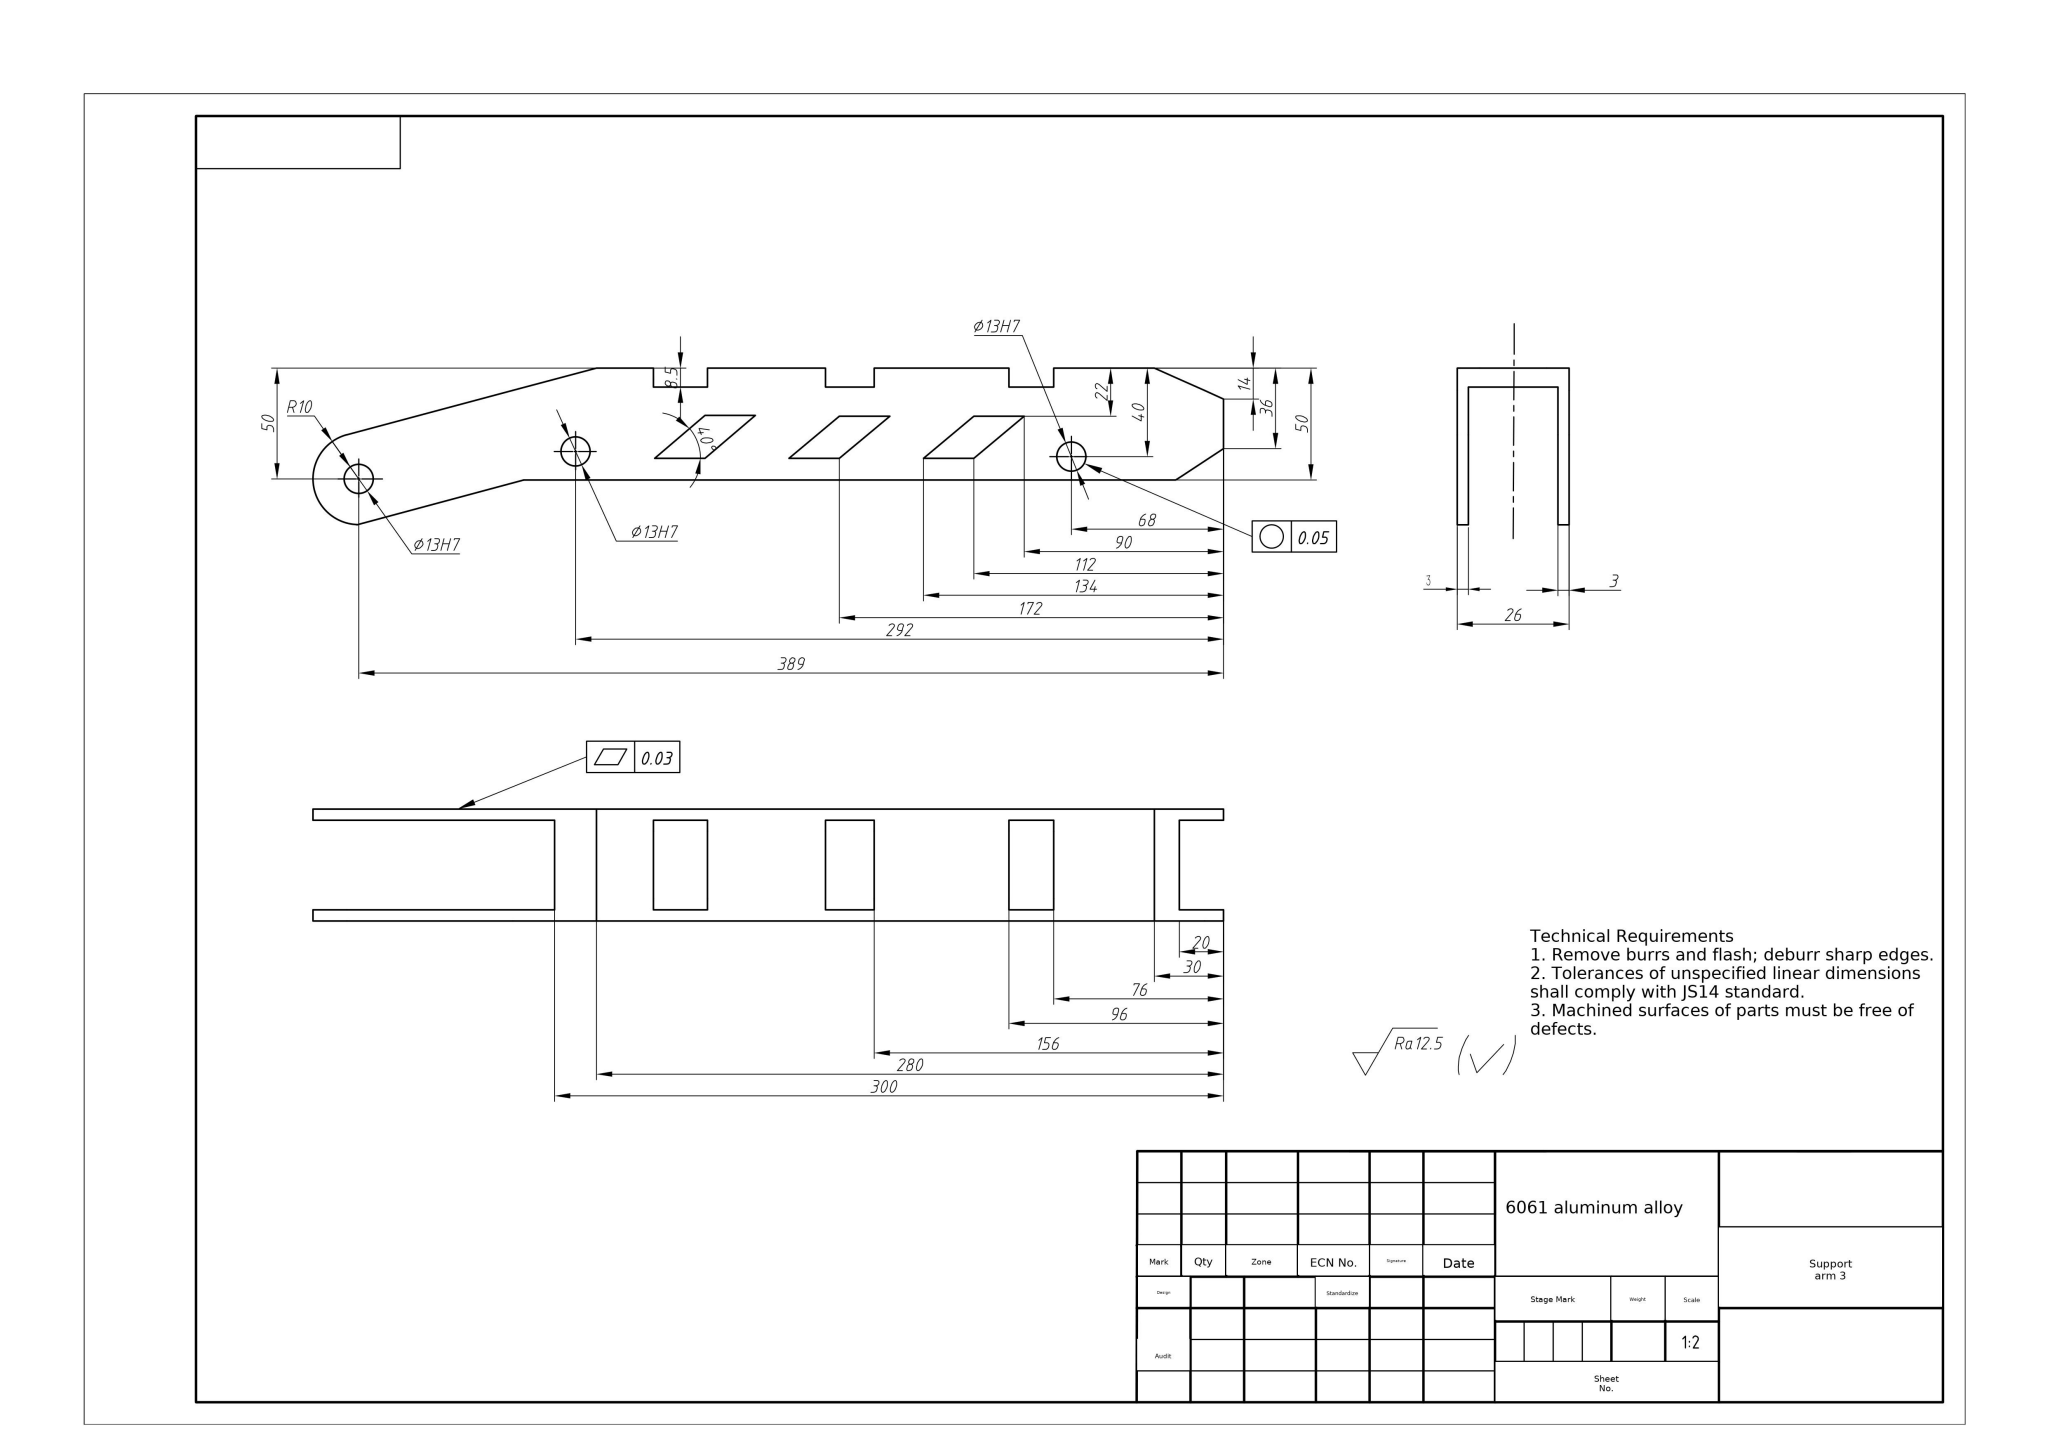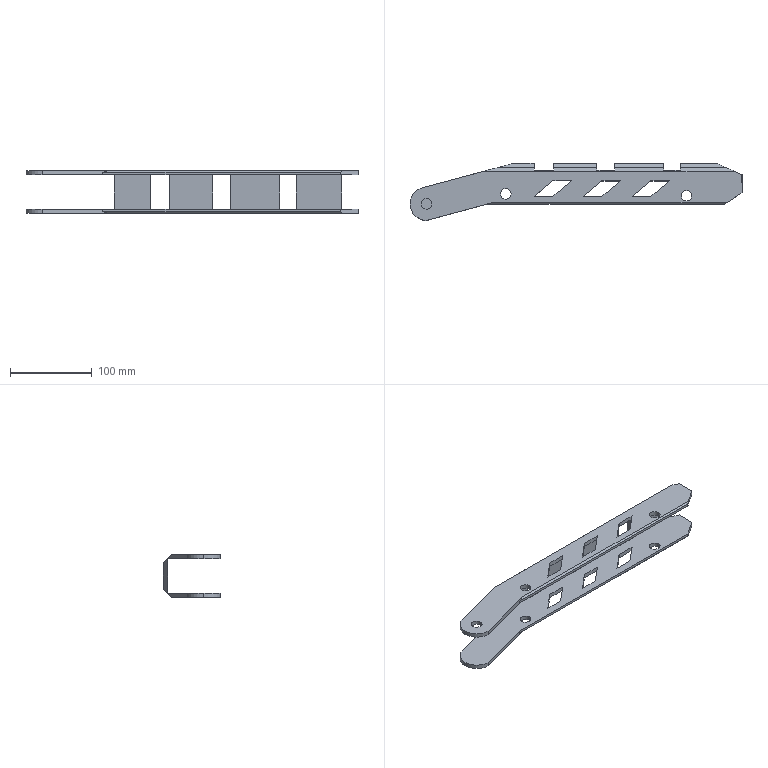Part | SolidWorks | mm | material 6061 aluminum alloy | 1 solid | 92 faces | box 406.54 x 69.92 x 52 mm | volume 186472 mm3 | plane 78 | cylinder 14 | commonest cylinder face diameters 13 x10 40.816 x4